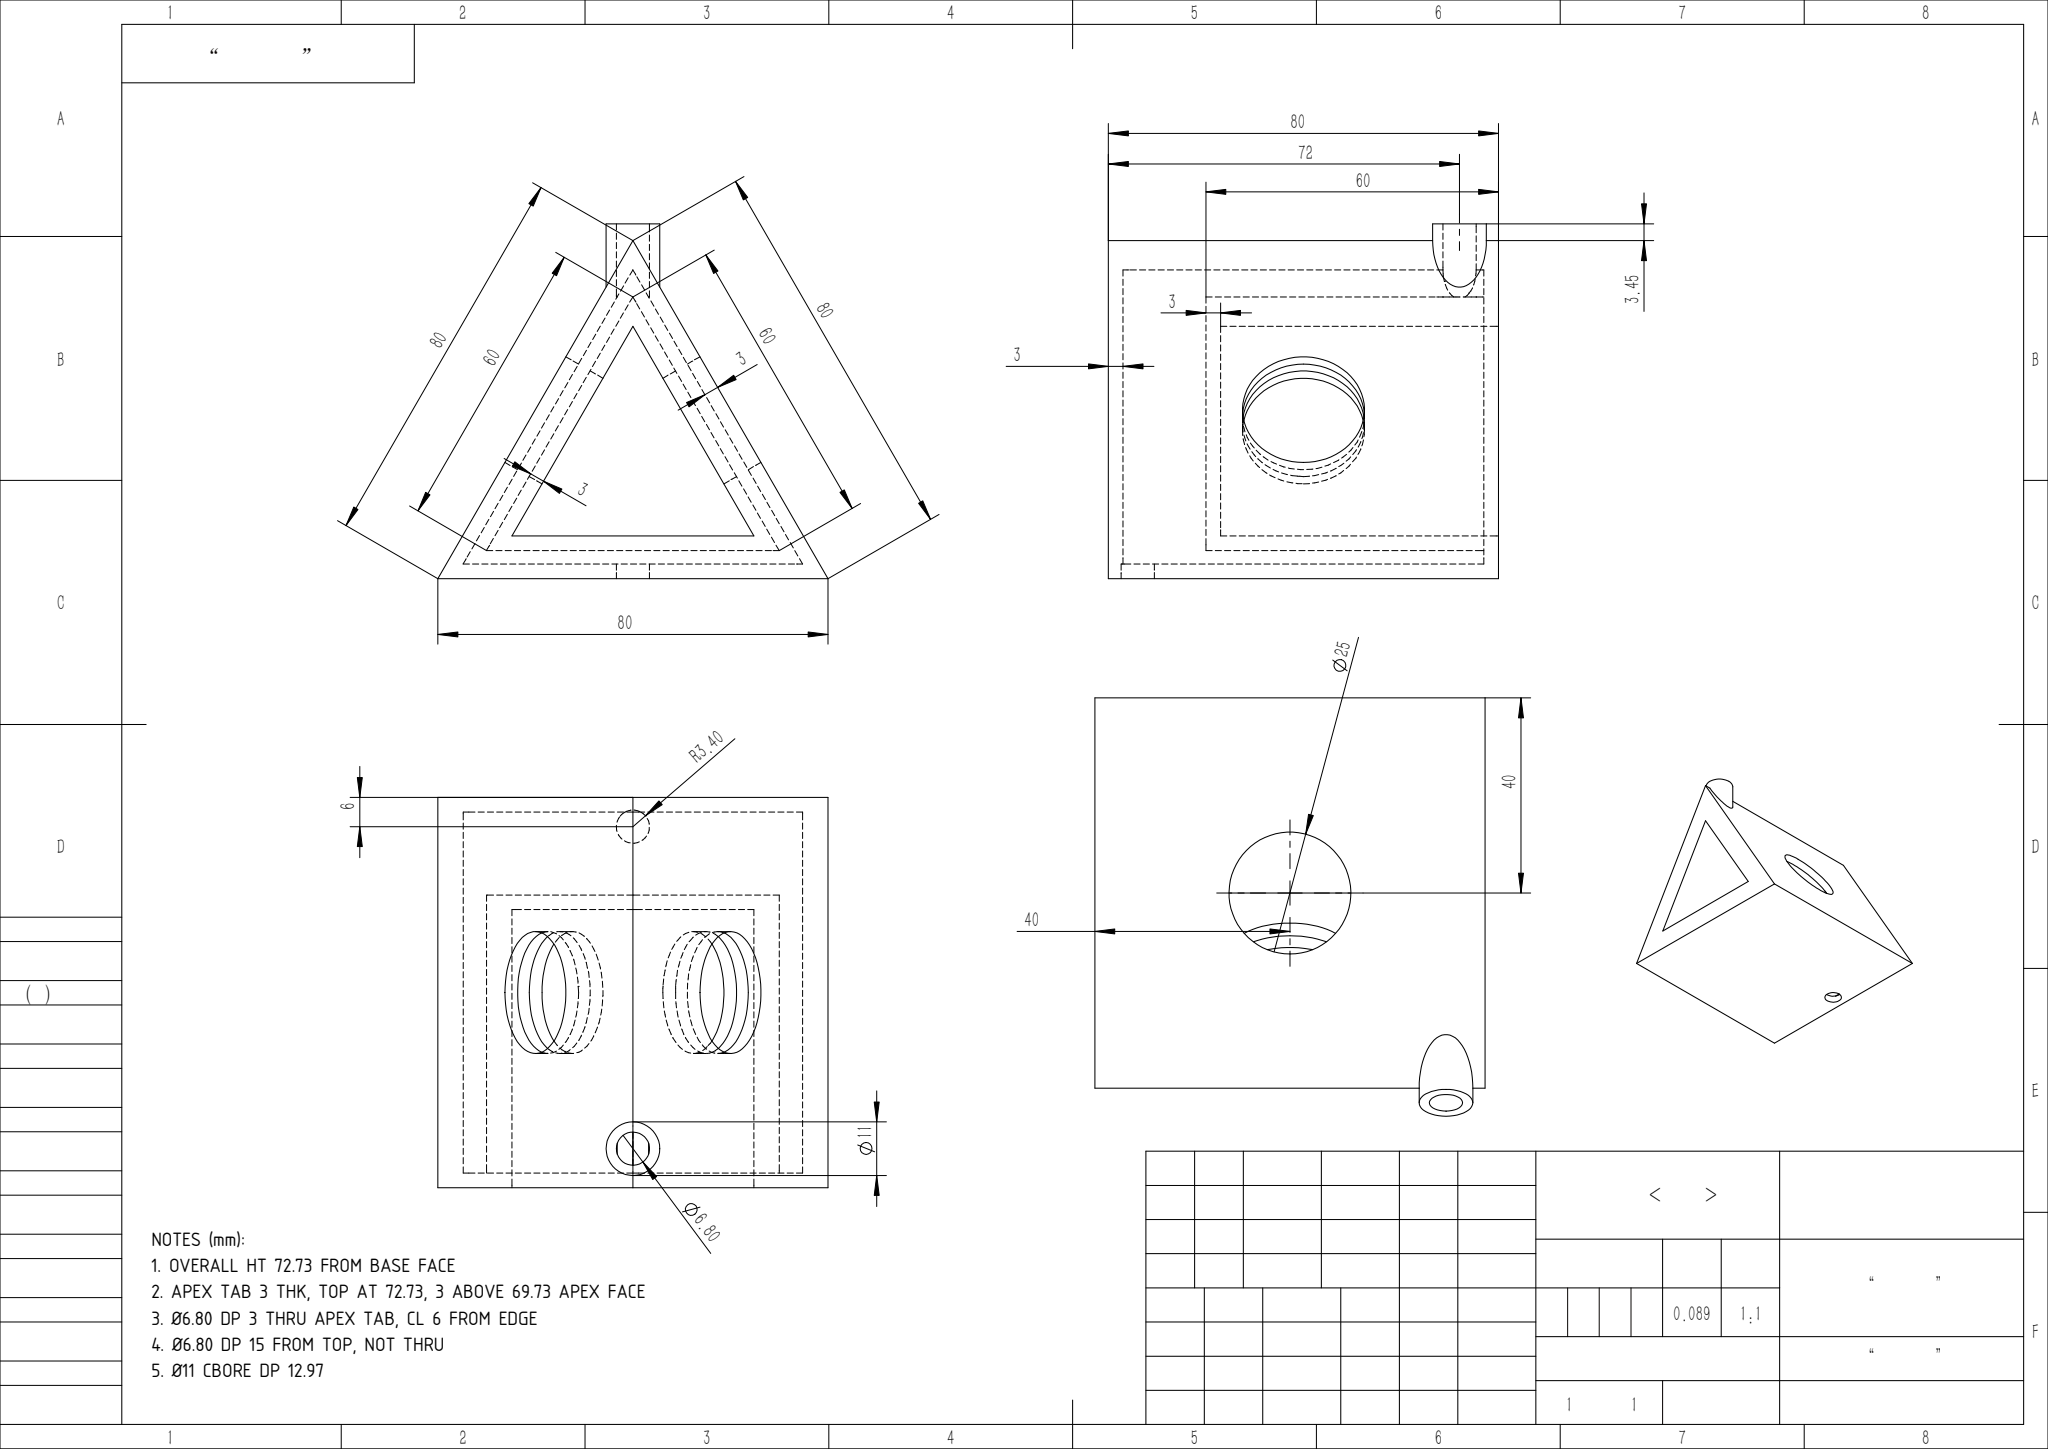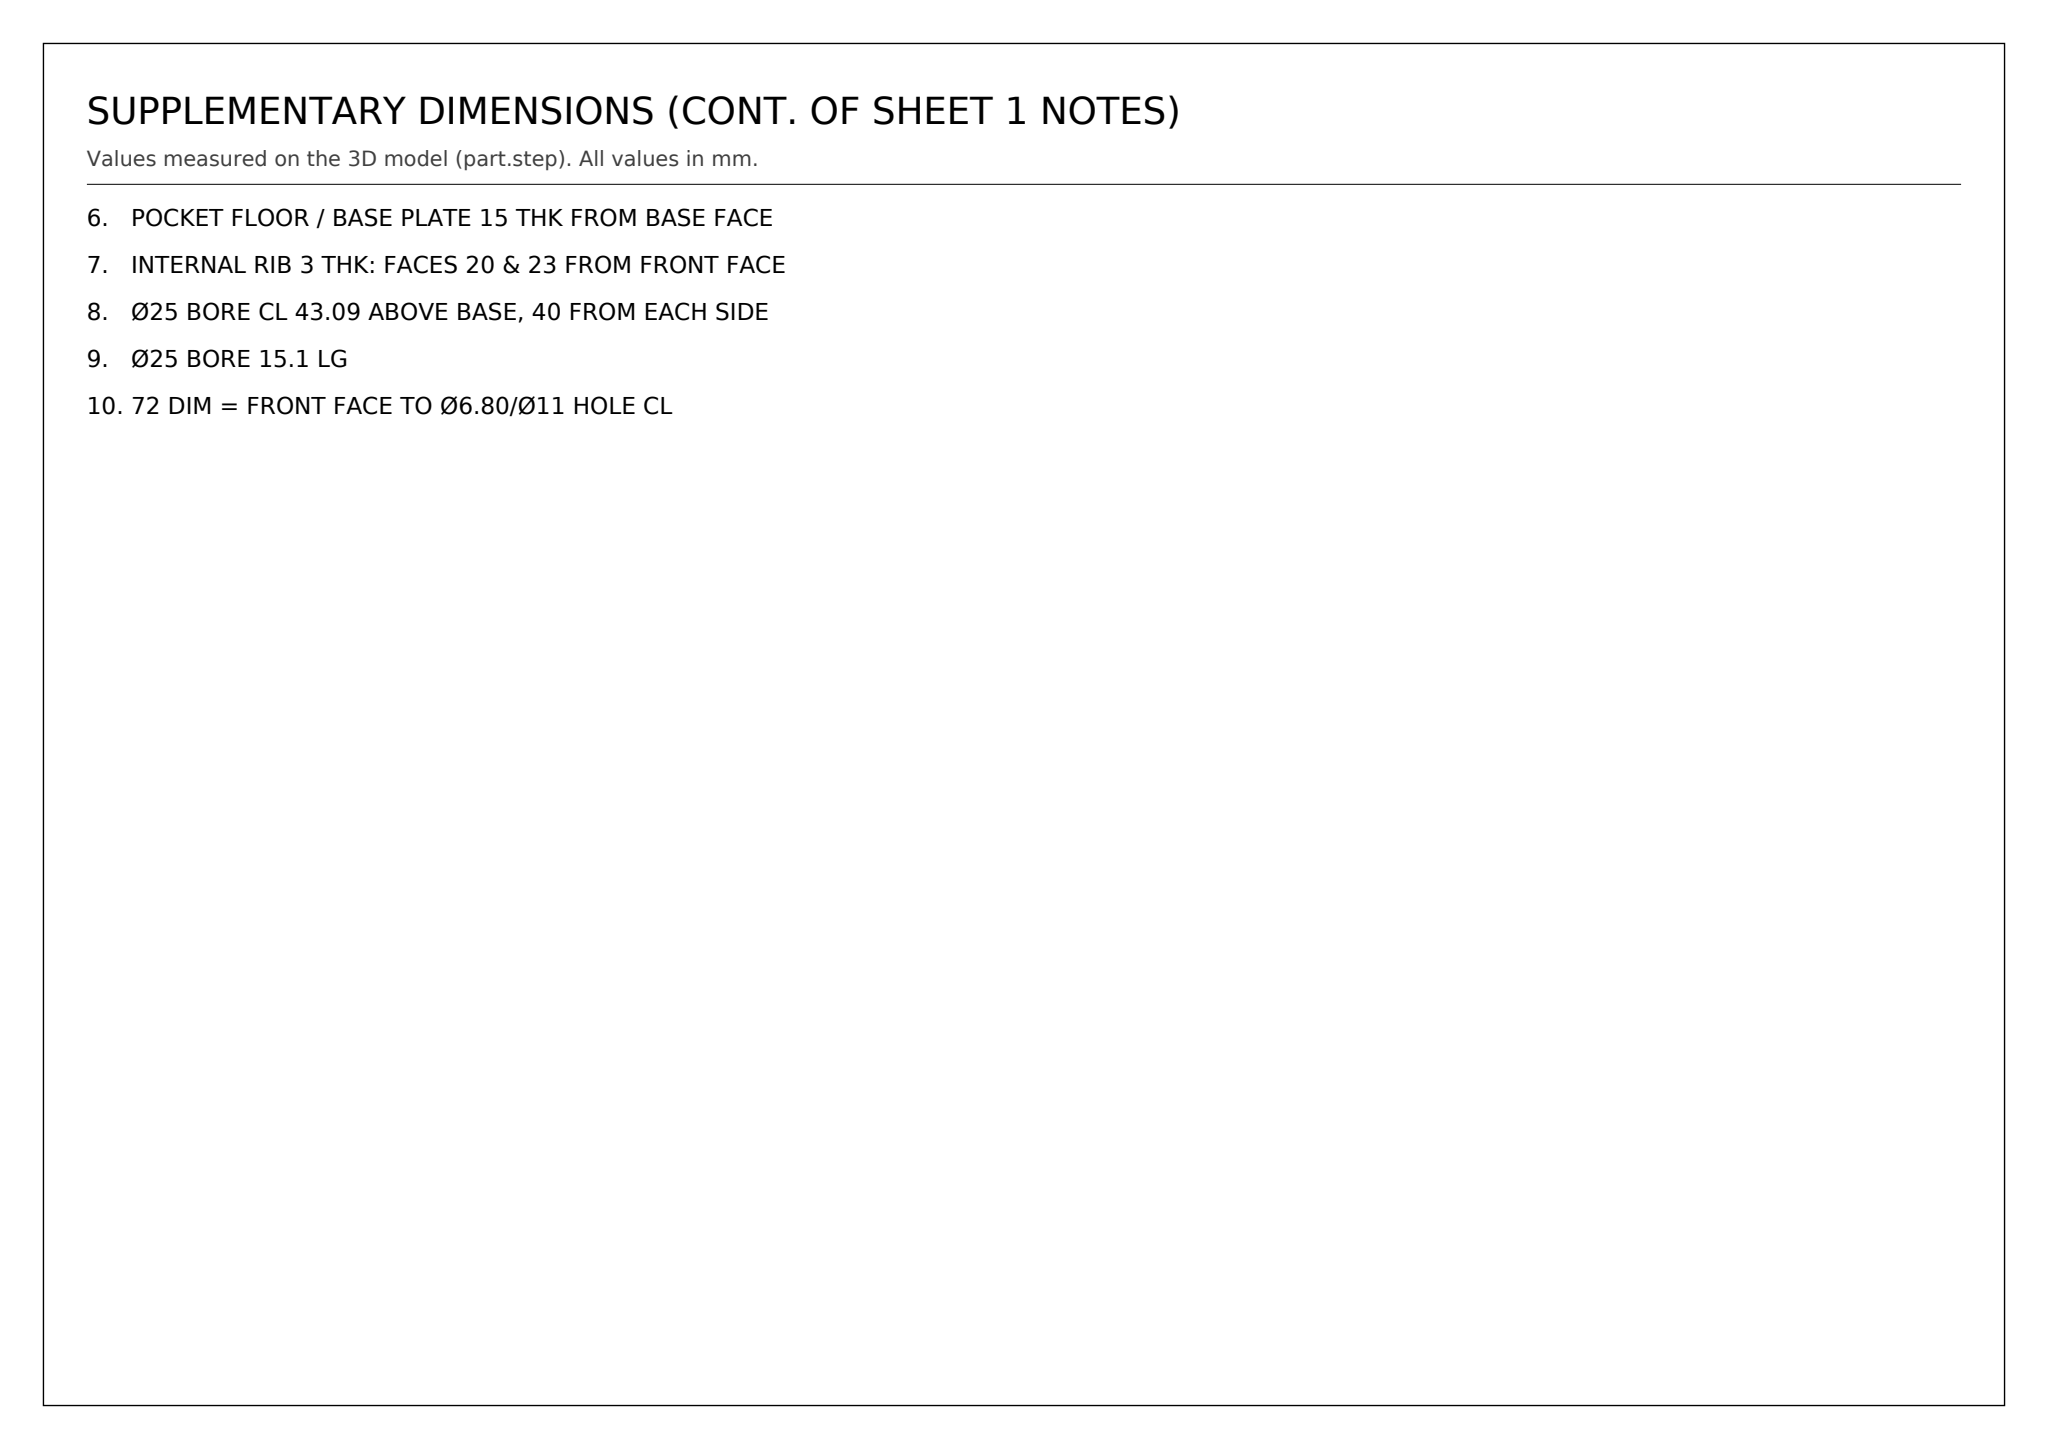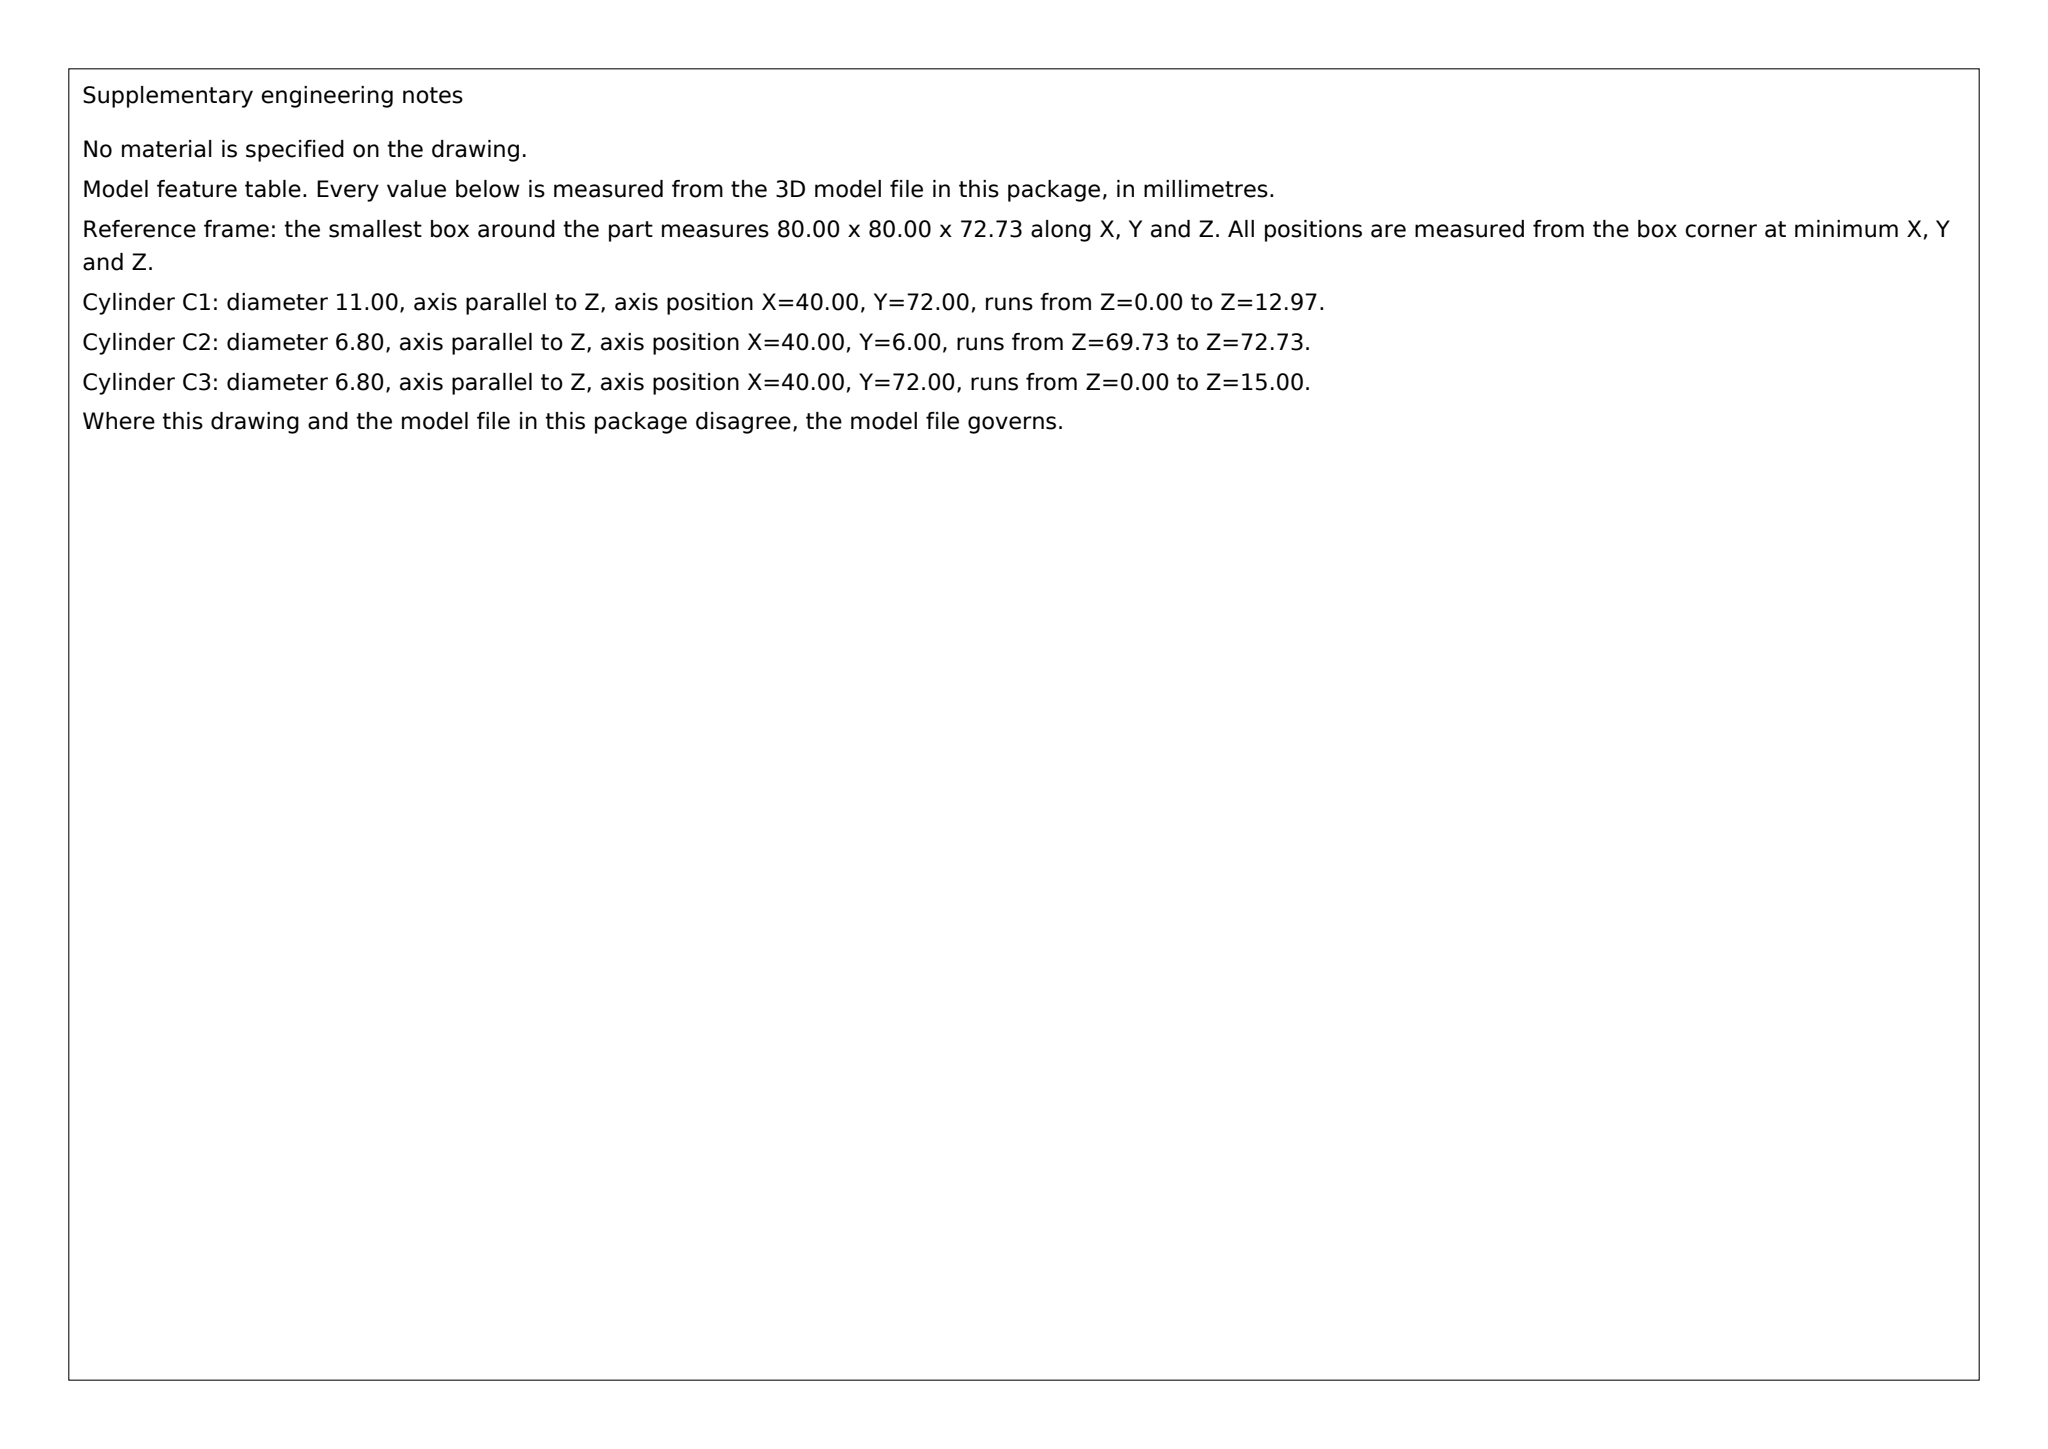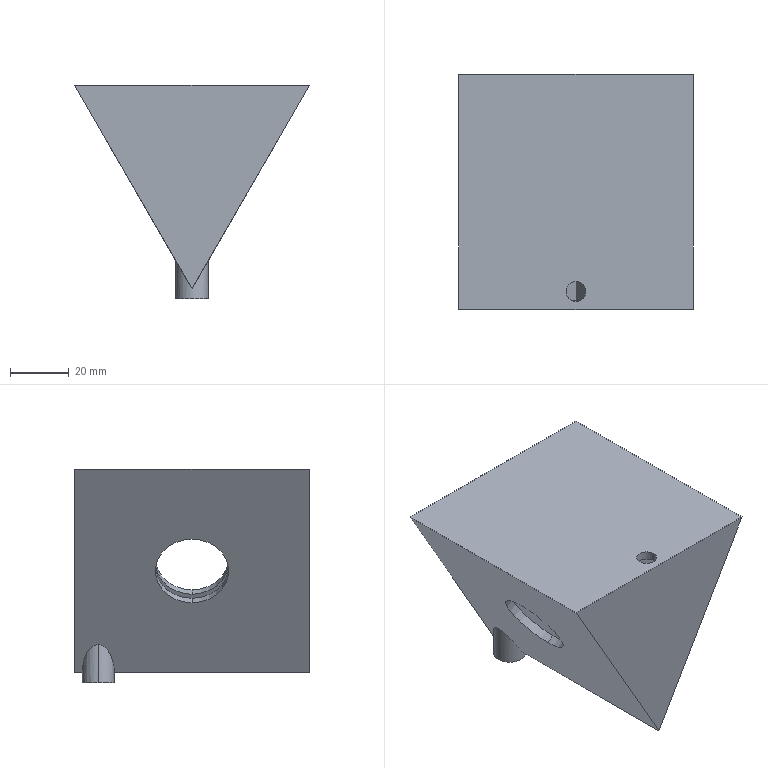Part | SolidWorks | mm | 1 solid | 39 faces | box 80 x 80 x 72.73 mm | volume 88840 mm3 | plane 23 | cylinder 16 | commonest cylinder face diameters 25 x8 6.8 x6 11 x2
Drawing notes:
OVERALL HT 72.73 FROM BASE FACE | from the solid: bbox_xyz z = 72.73; base plane z=0, top plane z=72.73
APEX TAB 3 THK, TOP AT 72.73, 3 ABOVE 69.73 APEX FACE | from the solid: axis_planes z=69.73 (apex face) and z=72.73 (tab top)
Ø6.80 DP 3 THRU APEX TAB, CL 6 FROM EDGE | from the solid: cylinder [6.8, z, (40.0, 6.0), len 3.0]
Ø6.80 DP 15 FROM TOP, NOT THRU | from the solid: cylinder [6.8, z, (40.0, 72.0), len 15.0]
Ø11 CBORE DP 12.97 | from the solid: cylinder [11.0, z, (40.0, 72.0), len 12.97]
POCKET FLOOR / BASE PLATE 15 THK FROM BASE FACE | from the solid: axis_planes z=15.0 (3 faces), base z=0
INTERNAL RIB 3 THK: FACES 20 & 23 FROM FRONT FACE | from the solid: axis_planes y=20.0 and y=23.0, front face y=0
Ø25 BORE CL 43.09 ABOVE BASE, 40 FROM EACH SIDE | from the solid: cylinder [25.0, x, (y=40.0, z=43.09)]
Ø25 BORE 15.1 LG | from the solid: cylinder [25.0, x, len 15.1]
72 DIM = FRONT FACE TO Ø6.80/Ø11 HOLE CL | from the solid: cylinders at y=72.0 from y=0 front face